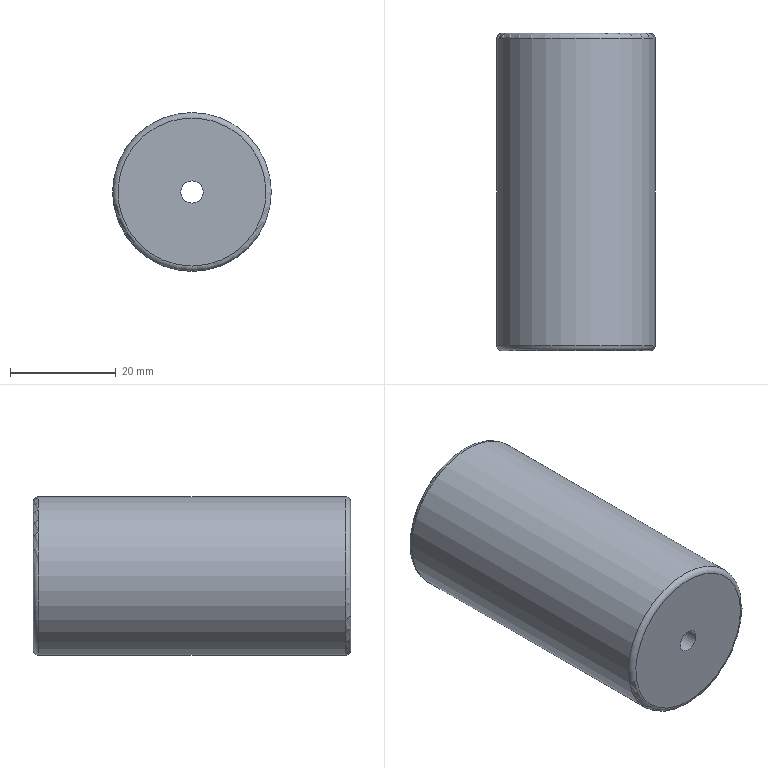Component | NX | 8_SLEEVE | 1 solid | 11 faces | box 30 x 60 x 30 mm | volume 28897 mm3 | plane 4 | cylinder 4 | torus 3 | commonest cylinder face diameters 30 x1 18 x1 20 x1 4.2 x1
STEP:
#1=CARTESIAN_POINT('',(0.,0.,0.));
#2=DIRECTION('',(0.,0.,1.));
#3=DIRECTION('',(1.,0.,0.));
#4=AXIS2_PLACEMENT_3D('',#1,#2,#3);
#5=CARTESIAN_POINT('',(-59.084,-92.206,-228.219));
#6=VERTEX_POINT('',#5);
#7=CARTESIAN_POINT('',(-59.084,-92.206,-238.219));
#8=DIRECTION('',(0.,-1.,0.));
#9=DIRECTION('',(0.,0.,1.));
#10=AXIS2_PLACEMENT_3D('',#7,#8,#9);
#11=CIRCLE('',#10,10.);
#12=CARTESIAN_POINT('',(-59.084,-92.206,-238.219));
#13=DIRECTION('',(0.,1.,0.));
#14=DIRECTION('',(0.,0.,1.));
#15=AXIS2_PLACEMENT_3D('',#12,#13,#14);
#16=PLANE('',#15);
#17=CARTESIAN_POINT('',(10.,0.));
#18=CARTESIAN_POINT('',(10.,-17.321));
#19=CARTESIAN_POINT('',(-5.,-8.66));
#20=CARTESIAN_POINT('',(-20.,-0.));
#21=CARTESIAN_POINT('',(-5.,8.66));
#22=CARTESIAN_POINT('',(10.,17.321));
#23=CARTESIAN_POINT('',(10.,0.));
#24=(BOUNDED_CURVE()B_SPLINE_CURVE(2,(#17,#18,#19,#20,#21,#22,#23),.UNSPECIFIED.,.T.,.F.)B_SPLINE_CURVE_WITH_KNOTS((1,2,2,2,2,1),(-2.094,0.,2.094,4.189,6.283,8.378),.UNSPECIFIED.)CURVE()GEOMETRIC_REPRESENTATION_ITEM()RATIONAL_B_SPLINE_CURVE((1.,0.5,1.,0.5,1.,0.5,1.))REPRESENTATION_ITEM(''));
#25=(GEOMETRIC_REPRESENTATION_CONTEXT(2)PARAMETRIC_REPRESENTATION_CONTEXT()REPRESENTATION_CONTEXT('',''));
#26=DEFINITIONAL_REPRESENTATION('',(#24),#25);
#27=PCURVE('',#16,#26);
#28=CARTESIAN_POINT('',(-59.084,-93.206,-238.219));
#29=DIRECTION('',(0.,1.,0.));
#30=DIRECTION('',(0.,0.,1.));
#31=AXIS2_PLACEMENT_3D('',#28,#29,#30);
#32=TOROIDAL_SURFACE('',#31,10.,1.);
#33=CARTESIAN_POINT('',(6.283,7.854));
#34=DIRECTION('',(-1.,0.));
#35=VECTOR('',#34,1.);
#36=LINE('',#33,#35);
#37=(GEOMETRIC_REPRESENTATION_CONTEXT(2)PARAMETRIC_REPRESENTATION_CONTEXT()REPRESENTATION_CONTEXT('',''));
#38=DEFINITIONAL_REPRESENTATION('',(#36),#37);
#39=PCURVE('',#32,#38);
#40=SURFACE_CURVE('',#11,(#27,#39),.PCURVE_S1.);
#41=EDGE_CURVE('',#6,#6,#40,.T.);
#42=ORIENTED_EDGE('',*,*,#41,.T.);
#43=EDGE_LOOP('',(#42));
#44=FACE_BOUND('',#43,.T.);
#45=CARTESIAN_POINT('',(-59.084,-92.206,-224.219));
#46=VERTEX_POINT('',#45);
#47=CARTESIAN_POINT('',(-59.084,-92.206,-238.219));
#48=DIRECTION('',(0.,1.,0.));
#49=DIRECTION('',(0.,0.,1.));
#50=AXIS2_PLACEMENT_3D('',#47,#48,#49);
#51=CIRCLE('',#50,14.);
#52=CARTESIAN_POINT('',(0.,0.));
#53=DIRECTION('',(1.,0.));
#54=AXIS2_PLACEMENT_2D('',#52,#53);
#55=CIRCLE('',#54,14.);
#56=(GEOMETRIC_REPRESENTATION_CONTEXT(2)PARAMETRIC_REPRESENTATION_CONTEXT()REPRESENTATION_CONTEXT('',''));
#57=DEFINITIONAL_REPRESENTATION('',(#55),#56);
#58=PCURVE('',#16,#57);
#59=CARTESIAN_POINT('',(-59.084,-93.206,-238.219));
#60=DIRECTION('',(0.,1.,0.));
#61=DIRECTION('',(0.,0.,1.));
#62=AXIS2_PLACEMENT_3D('',#59,#60,#61);
#63=TOROIDAL_SURFACE('',#62,14.,1.);
#64=CARTESIAN_POINT('',(0.,7.854));
#65=DIRECTION('',(1.,0.));
#66=VECTOR('',#65,1.);
#67=LINE('',#64,#66);
#68=(GEOMETRIC_REPRESENTATION_CONTEXT(2)PARAMETRIC_REPRESENTATION_CONTEXT()REPRESENTATION_CONTEXT('',''));
#69=DEFINITIONAL_REPRESENTATION('',(#67),#68);
#70=PCURVE('',#63,#69);
#71=SURFACE_CURVE('',#51,(#58,#70),.PCURVE_S1.);
#72=EDGE_CURVE('',#46,#46,#71,.T.);
#73=ORIENTED_EDGE('',*,*,#72,.T.);
#74=EDGE_LOOP('',(#73));
#75=FACE_BOUND('',#74,.T.);
#76=ADVANCED_FACE('',(#44,#75),#16,.T.);
#77=CARTESIAN_POINT('',(-59.084,-152.206,-252.219));
#78=VERTEX_POINT('',#77);
#79=CARTESIAN_POINT('',(-59.084,-152.206,-238.219));
#80=DIRECTION('',(0.,-1.,0.));
#81=DIRECTION('',(0.,0.,-1.));
#82=AXIS2_PLACEMENT_3D('',#79,#80,#81);
#83=CIRCLE('',#82,14.);
#84=CARTESIAN_POINT('',(-59.084,-152.206,-238.219));
#85=DIRECTION('',(0.,-1.,0.));
#86=DIRECTION('',(0.,0.,-1.));
#87=AXIS2_PLACEMENT_3D('',#84,#85,#86);
#88=PLANE('',#87);
#89=CARTESIAN_POINT('',(0.,0.));
#90=DIRECTION('',(1.,0.));
#91=AXIS2_PLACEMENT_2D('',#89,#90);
#92=CIRCLE('',#91,14.);
#93=(GEOMETRIC_REPRESENTATION_CONTEXT(2)PARAMETRIC_REPRESENTATION_CONTEXT()REPRESENTATION_CONTEXT('',''));
#94=DEFINITIONAL_REPRESENTATION('',(#92),#93);
#95=PCURVE('',#88,#94);
#96=CARTESIAN_POINT('',(-59.084,-151.206,-238.219));
#97=DIRECTION('',(0.,-1.,0.));
#98=DIRECTION('',(0.,0.,-1.));
#99=AXIS2_PLACEMENT_3D('',#96,#97,#98);
#100=TOROIDAL_SURFACE('',#99,14.,1.);
#101=CARTESIAN_POINT('',(0.,7.854));
#102=DIRECTION('',(1.,0.));
#103=VECTOR('',#102,1.);
#104=LINE('',#101,#103);
#105=(GEOMETRIC_REPRESENTATION_CONTEXT(2)PARAMETRIC_REPRESENTATION_CONTEXT()REPRESENTATION_CONTEXT('',''));
#106=DEFINITIONAL_REPRESENTATION('',(#104),#105);
#107=PCURVE('',#100,#106);
#108=SURFACE_CURVE('',#83,(#95,#107),.PCURVE_S1.);
#109=EDGE_CURVE('',#78,#78,#108,.T.);
#110=ORIENTED_EDGE('',*,*,#109,.T.);
#111=EDGE_LOOP('',(#110));
#112=FACE_BOUND('',#111,.T.);
#113=CARTESIAN_POINT('',(-59.084,-152.206,-236.119));
#114=VERTEX_POINT('',#113);
#115=CARTESIAN_POINT('',(-59.084,-152.206,-238.219));
#116=DIRECTION('',(0.,1.,0.));
#117=DIRECTION('',(0.,0.,1.));
#118=AXIS2_PLACEMENT_3D('',#115,#116,#117);
#119=CIRCLE('',#118,2.1);
#120=CARTESIAN_POINT('',(-2.1,0.));
#121=CARTESIAN_POINT('',(-2.1,3.637));
#122=CARTESIAN_POINT('',(1.05,1.819));
#123=CARTESIAN_POINT('',(4.2,0.));
#124=CARTESIAN_POINT('',(1.05,-1.819));
#125=CARTESIAN_POINT('',(-2.1,-3.637));
#126=CARTESIAN_POINT('',(-2.1,0.));
#127=(BOUNDED_CURVE()B_SPLINE_CURVE(2,(#120,#121,#122,#123,#124,#125,#126),.UNSPECIFIED.,.T.,.F.)B_SPLINE_CURVE_WITH_KNOTS((1,2,2,2,2,1),(-2.094,0.,2.094,4.189,6.283,8.378),.UNSPECIFIED.)CURVE()GEOMETRIC_REPRESENTATION_ITEM()RATIONAL_B_SPLINE_CURVE((1.,0.5,1.,0.5,1.,0.5,1.))REPRESENTATION_ITEM(''));
#128=(GEOMETRIC_REPRESENTATION_CONTEXT(2)PARAMETRIC_REPRESENTATION_CONTEXT()REPRESENTATION_CONTEXT('',''));
#129=DEFINITIONAL_REPRESENTATION('',(#127),#128);
#130=PCURVE('',#88,#129);
#131=CARTESIAN_POINT('',(-59.084,-152.206,-238.219));
#132=DIRECTION('',(0.,1.,0.));
#133=DIRECTION('',(0.,0.,1.));
#134=AXIS2_PLACEMENT_3D('',#131,#132,#133);
#135=CYLINDRICAL_SURFACE('',#134,2.1);
#136=CARTESIAN_POINT('',(0.,0.));
#137=DIRECTION('',(1.,0.));
#138=VECTOR('',#137,1.);
#139=LINE('',#136,#138);
#140=(GEOMETRIC_REPRESENTATION_CONTEXT(2)PARAMETRIC_REPRESENTATION_CONTEXT()REPRESENTATION_CONTEXT('',''));
#141=DEFINITIONAL_REPRESENTATION('',(#139),#140);
#142=PCURVE('',#135,#141);
#143=SURFACE_CURVE('',#119,(#130,#142),.PCURVE_S1.);
#144=EDGE_CURVE('',#114,#114,#143,.T.);
#145=ORIENTED_EDGE('',*,*,#144,.T.);
#146=EDGE_LOOP('',(#145));
#147=FACE_BOUND('',#146,.T.);
#148=ADVANCED_FACE('',(#112,#147),#88,.T.);
#149=CARTESIAN_POINT('',(-59.084,-93.206,-223.219));
#150=VERTEX_POINT('',#149);
#151=CARTESIAN_POINT('',(-59.084,-93.206,-238.219));
#152=DIRECTION('',(0.,-1.,0.));
#153=DIRECTION('',(0.,0.,1.));
#154=AXIS2_PLACEMENT_3D('',#151,#152,#153);
#155=CIRCLE('',#154,15.);
#156=CARTESIAN_POINT('',(-59.084,-152.206,-238.219));
#157=DIRECTION('',(0.,1.,0.));
#158=DIRECTION('',(0.,0.,1.));
#159=AXIS2_PLACEMENT_3D('',#156,#157,#158);
#160=CYLINDRICAL_SURFACE('',#159,15.);
#161=CARTESIAN_POINT('',(6.283,59.));
#162=DIRECTION('',(-1.,0.));
#163=VECTOR('',#162,1.);
#164=LINE('',#161,#163);
#165=(GEOMETRIC_REPRESENTATION_CONTEXT(2)PARAMETRIC_REPRESENTATION_CONTEXT()REPRESENTATION_CONTEXT('',''));
#166=DEFINITIONAL_REPRESENTATION('',(#164),#165);
#167=PCURVE('',#160,#166);
#168=CARTESIAN_POINT('',(6.283,6.283));
#169=DIRECTION('',(-1.,0.));
#170=VECTOR('',#169,1.);
#171=LINE('',#168,#170);
#172=(GEOMETRIC_REPRESENTATION_CONTEXT(2)PARAMETRIC_REPRESENTATION_CONTEXT()REPRESENTATION_CONTEXT('',''));
#173=DEFINITIONAL_REPRESENTATION('',(#171),#172);
#174=PCURVE('',#63,#173);
#175=SURFACE_CURVE('',#155,(#167,#174),.PCURVE_S1.);
#176=EDGE_CURVE('',#150,#150,#175,.T.);
#177=ORIENTED_EDGE('',*,*,#176,.T.);
#178=CARTESIAN_POINT('',(-59.084,-151.206,-223.219));
#179=VERTEX_POINT('',#178);
#180=CARTESIAN_POINT('',(-59.084,-151.206,-223.219));
#181=CARTESIAN_POINT('',(-59.084,-93.206,-223.219));
#182=B_SPLINE_CURVE_WITH_KNOTS('',1,(#180,#181),.UNSPECIFIED.,.F.,.F.,(2,2),(1.,59.),.PIECEWISE_BEZIER_KNOTS.);
#183=CARTESIAN_POINT('',(0.,0.));
#184=DIRECTION('',(0.,1.));
#185=VECTOR('',#184,1.);
#186=LINE('',#183,#185);
#187=(GEOMETRIC_REPRESENTATION_CONTEXT(2)PARAMETRIC_REPRESENTATION_CONTEXT()REPRESENTATION_CONTEXT('',''));
#188=DEFINITIONAL_REPRESENTATION('',(#186),#187);
#189=PCURVE('',#160,#188);
#190=CARTESIAN_POINT('',(6.283,0.));
#191=DIRECTION('',(0.,1.));
#192=VECTOR('',#191,1.);
#193=LINE('',#190,#192);
#194=(GEOMETRIC_REPRESENTATION_CONTEXT(2)PARAMETRIC_REPRESENTATION_CONTEXT()REPRESENTATION_CONTEXT('',''));
#195=DEFINITIONAL_REPRESENTATION('',(#193),#194);
#196=PCURVE('',#160,#195);
#197=SEAM_CURVE('',#182,(#189,#196),.PCURVE_S1.);
#198=EDGE_CURVE('',#179,#150,#197,.T.);
#199=ORIENTED_EDGE('',*,*,#198,.F.);
#200=CARTESIAN_POINT('',(-59.084,-151.206,-253.219));
#201=VERTEX_POINT('',#200);
#202=CARTESIAN_POINT('',(-59.084,-151.206,-238.219));
#203=DIRECTION('',(0.,1.,0.));
#204=DIRECTION('',(0.,0.,-1.));
#205=AXIS2_PLACEMENT_3D('',#202,#203,#204);
#206=CIRCLE('',#205,15.);
#207=CARTESIAN_POINT('',(-3.142,1.));
#208=DIRECTION('',(1.,0.));
#209=VECTOR('',#208,1.);
#210=LINE('',#207,#209);
#211=(GEOMETRIC_REPRESENTATION_CONTEXT(2)PARAMETRIC_REPRESENTATION_CONTEXT()REPRESENTATION_CONTEXT('',''));
#212=DEFINITIONAL_REPRESENTATION('',(#210),#211);
#213=PCURVE('',#160,#212);
#214=CARTESIAN_POINT('',(6.283,6.283));
#215=DIRECTION('',(-1.,0.));
#216=VECTOR('',#215,1.);
#217=LINE('',#214,#216);
#218=(GEOMETRIC_REPRESENTATION_CONTEXT(2)PARAMETRIC_REPRESENTATION_CONTEXT()REPRESENTATION_CONTEXT('',''));
#219=DEFINITIONAL_REPRESENTATION('',(#217),#218);
#220=PCURVE('',#100,#219);
#221=SURFACE_CURVE('',#206,(#213,#220),.PCURVE_S1.);
#222=EDGE_CURVE('',#179,#201,#221,.T.);
#223=ORIENTED_EDGE('',*,*,#222,.T.);
#224=CARTESIAN_POINT('',(-59.084,-151.206,-238.219));
#225=DIRECTION('',(0.,1.,0.));
#226=DIRECTION('',(0.,0.,-1.));
#227=AXIS2_PLACEMENT_3D('',#224,#225,#226);
#228=CIRCLE('',#227,15.);
#229=CARTESIAN_POINT('',(3.142,1.));
#230=DIRECTION('',(1.,0.));
#231=VECTOR('',#230,1.);
#232=LINE('',#229,#231);
#233=(GEOMETRIC_REPRESENTATION_CONTEXT(2)PARAMETRIC_REPRESENTATION_CONTEXT()REPRESENTATION_CONTEXT('',''));
#234=DEFINITIONAL_REPRESENTATION('',(#232),#233);
#235=PCURVE('',#160,#234);
#236=CARTESIAN_POINT('',(6.283,6.283));
#237=DIRECTION('',(-1.,0.));
#238=VECTOR('',#237,1.);
#239=LINE('',#236,#238);
#240=(GEOMETRIC_REPRESENTATION_CONTEXT(2)PARAMETRIC_REPRESENTATION_CONTEXT()REPRESENTATION_CONTEXT('',''));
#241=DEFINITIONAL_REPRESENTATION('',(#239),#240);
#242=PCURVE('',#100,#241);
#243=SURFACE_CURVE('',#228,(#235,#242),.PCURVE_S1.);
#244=EDGE_CURVE('',#201,#179,#243,.T.);
#245=ORIENTED_EDGE('',*,*,#244,.T.);
#246=ORIENTED_EDGE('',*,*,#198,.T.);
#247=EDGE_LOOP('',(#177,#199,#223,#245,#246));
#248=FACE_BOUND('',#247,.T.);
#249=ADVANCED_FACE('',(#248),#160,.T.);
#250=CARTESIAN_POINT('',(-59.084,-93.206,-229.219));
#251=VERTEX_POINT('',#250);
#252=CARTESIAN_POINT('',(-59.084,-93.206,-238.219));
#253=DIRECTION('',(0.,1.,0.));
#254=DIRECTION('',(0.,0.,1.));
#255=AXIS2_PLACEMENT_3D('',#252,#253,#254);
#256=CIRCLE('',#255,9.);
#257=CARTESIAN_POINT('',(-59.084,-92.206,-238.219));
#258=DIRECTION('',(0.,-1.,0.));
#259=DIRECTION('',(0.,0.,1.));
#260=AXIS2_PLACEMENT_3D('',#257,#258,#259);
#261=CYLINDRICAL_SURFACE('',#260,9.);
#262=CARTESIAN_POINT('',(6.283,1.));
#263=DIRECTION('',(-1.,0.));
#264=VECTOR('',#263,1.);
#265=LINE('',#262,#264);
#266=(GEOMETRIC_REPRESENTATION_CONTEXT(2)PARAMETRIC_REPRESENTATION_CONTEXT()REPRESENTATION_CONTEXT('',''));
#267=DEFINITIONAL_REPRESENTATION('',(#265),#266);
#268=PCURVE('',#261,#267);
#269=CARTESIAN_POINT('',(0.,9.425));
#270=DIRECTION('',(1.,0.));
#271=VECTOR('',#270,1.);
#272=LINE('',#269,#271);
#273=(GEOMETRIC_REPRESENTATION_CONTEXT(2)PARAMETRIC_REPRESENTATION_CONTEXT()REPRESENTATION_CONTEXT('',''));
#274=DEFINITIONAL_REPRESENTATION('',(#272),#273);
#275=PCURVE('',#32,#274);
#276=SURFACE_CURVE('',#256,(#268,#275),.PCURVE_S1.);
#277=EDGE_CURVE('',#251,#251,#276,.T.);
#278=ORIENTED_EDGE('',*,*,#277,.F.);
#279=CARTESIAN_POINT('',(-59.084,-142.206,-229.219));
#280=VERTEX_POINT('',#279);
#281=CARTESIAN_POINT('',(-59.084,-93.206,-229.219));
#282=CARTESIAN_POINT('',(-59.084,-142.206,-229.219));
#283=B_SPLINE_CURVE_WITH_KNOTS('',1,(#281,#282),.UNSPECIFIED.,.F.,.F.,(2,2),(1.,50.),.PIECEWISE_BEZIER_KNOTS.);
#284=CARTESIAN_POINT('',(6.283,0.));
#285=DIRECTION('',(0.,1.));
#286=VECTOR('',#285,1.);
#287=LINE('',#284,#286);
#288=(GEOMETRIC_REPRESENTATION_CONTEXT(2)PARAMETRIC_REPRESENTATION_CONTEXT()REPRESENTATION_CONTEXT('',''));
#289=DEFINITIONAL_REPRESENTATION('',(#287),#288);
#290=PCURVE('',#261,#289);
#291=CARTESIAN_POINT('',(0.,0.));
#292=DIRECTION('',(0.,1.));
#293=VECTOR('',#292,1.);
#294=LINE('',#291,#293);
#295=(GEOMETRIC_REPRESENTATION_CONTEXT(2)PARAMETRIC_REPRESENTATION_CONTEXT()REPRESENTATION_CONTEXT('',''));
#296=DEFINITIONAL_REPRESENTATION('',(#294),#295);
#297=PCURVE('',#261,#296);
#298=SEAM_CURVE('',#283,(#290,#297),.PCURVE_S1.);
#299=EDGE_CURVE('',#251,#280,#298,.T.);
#300=ORIENTED_EDGE('',*,*,#299,.T.);
#301=CARTESIAN_POINT('',(-59.084,-142.206,-238.219));
#302=DIRECTION('',(0.,-1.,0.));
#303=DIRECTION('',(0.,0.,1.));
#304=AXIS2_PLACEMENT_3D('',#301,#302,#303);
#305=CIRCLE('',#304,9.);
#306=CARTESIAN_POINT('',(0.,50.));
#307=DIRECTION('',(1.,0.));
#308=VECTOR('',#307,1.);
#309=LINE('',#306,#308);
#310=(GEOMETRIC_REPRESENTATION_CONTEXT(2)PARAMETRIC_REPRESENTATION_CONTEXT()REPRESENTATION_CONTEXT('',''));
#311=DEFINITIONAL_REPRESENTATION('',(#309),#310);
#312=PCURVE('',#261,#311);
#313=CARTESIAN_POINT('',(-59.084,-142.206,-238.219));
#314=DIRECTION('',(0.,1.,0.));
#315=DIRECTION('',(0.,0.,1.));
#316=AXIS2_PLACEMENT_3D('',#313,#314,#315);
#317=PLANE('',#316);
#318=CARTESIAN_POINT('',(9.,0.));
#319=CARTESIAN_POINT('',(9.,-15.588));
#320=CARTESIAN_POINT('',(-4.5,-7.794));
#321=CARTESIAN_POINT('',(-18.,-0.));
#322=CARTESIAN_POINT('',(-4.5,7.794));
#323=CARTESIAN_POINT('',(9.,15.588));
#324=CARTESIAN_POINT('',(9.,0.));
#325=(BOUNDED_CURVE()B_SPLINE_CURVE(2,(#318,#319,#320,#321,#322,#323,#324),.UNSPECIFIED.,.T.,.F.)B_SPLINE_CURVE_WITH_KNOTS((1,2,2,2,2,1),(-2.094,0.,2.094,4.189,6.283,8.378),.UNSPECIFIED.)CURVE()GEOMETRIC_REPRESENTATION_ITEM()RATIONAL_B_SPLINE_CURVE((1.,0.5,1.,0.5,1.,0.5,1.))REPRESENTATION_ITEM(''));
#326=(GEOMETRIC_REPRESENTATION_CONTEXT(2)PARAMETRIC_REPRESENTATION_CONTEXT()REPRESENTATION_CONTEXT('',''));
#327=DEFINITIONAL_REPRESENTATION('',(#325),#326);
#328=PCURVE('',#317,#327);
#329=SURFACE_CURVE('',#305,(#312,#328),.PCURVE_S1.);
#330=EDGE_CURVE('',#280,#280,#329,.T.);
#331=ORIENTED_EDGE('',*,*,#330,.F.);
#332=ORIENTED_EDGE('',*,*,#299,.F.);
#333=EDGE_LOOP('',(#278,#300,#331,#332));
#334=FACE_BOUND('',#333,.F.);
#335=ADVANCED_FACE('',(#334),#261,.F.);
#336=CARTESIAN_POINT('',(-59.084,-142.206,-228.219));
#337=VERTEX_POINT('',#336);
#338=CARTESIAN_POINT('',(-59.084,-142.206,-238.219));
#339=DIRECTION('',(0.,1.,0.));
#340=DIRECTION('',(0.,0.,1.));
#341=AXIS2_PLACEMENT_3D('',#338,#339,#340);
#342=CIRCLE('',#341,10.);
#343=CARTESIAN_POINT('',(0.,0.));
#344=DIRECTION('',(1.,0.));
#345=AXIS2_PLACEMENT_2D('',#343,#344);
#346=CIRCLE('',#345,10.);
#347=(GEOMETRIC_REPRESENTATION_CONTEXT(2)PARAMETRIC_REPRESENTATION_CONTEXT()REPRESENTATION_CONTEXT('',''));
#348=DEFINITIONAL_REPRESENTATION('',(#346),#347);
#349=PCURVE('',#317,#348);
#350=CARTESIAN_POINT('',(-59.084,-142.206,-238.219));
#351=DIRECTION('',(0.,-1.,0.));
#352=DIRECTION('',(0.,0.,1.));
#353=AXIS2_PLACEMENT_3D('',#350,#351,#352);
#354=CYLINDRICAL_SURFACE('',#353,10.);
#355=CARTESIAN_POINT('',(6.283,0.));
#356=DIRECTION('',(-1.,0.));
#357=VECTOR('',#356,1.);
#358=LINE('',#355,#357);
#359=(GEOMETRIC_REPRESENTATION_CONTEXT(2)PARAMETRIC_REPRESENTATION_CONTEXT()REPRESENTATION_CONTEXT('',''));
#360=DEFINITIONAL_REPRESENTATION('',(#358),#359);
#361=PCURVE('',#354,#360);
#362=SURFACE_CURVE('',#342,(#349,#361),.PCURVE_S1.);
#363=EDGE_CURVE('',#337,#337,#362,.T.);
#364=ORIENTED_EDGE('',*,*,#363,.F.);
#365=EDGE_LOOP('',(#364));
#366=FACE_BOUND('',#365,.T.);
#367=ORIENTED_EDGE('',*,*,#330,.F.);
#368=EDGE_LOOP('',(#367));
#369=FACE_BOUND('',#368,.T.);
#370=ADVANCED_FACE('',(#366,#369),#317,.F.);
#371=CARTESIAN_POINT('',(-59.084,-144.206,-240.319));
#372=VERTEX_POINT('',#371);
#373=CARTESIAN_POINT('',(-59.084,-144.206,-236.119));
#374=VERTEX_POINT('',#373);
#375=CARTESIAN_POINT('',(-59.084,-144.206,-238.219));
#376=DIRECTION('',(0.,-1.,0.));
#377=DIRECTION('',(0.,0.,-1.));
#378=AXIS2_PLACEMENT_3D('',#375,#376,#377);
#379=CIRCLE('',#378,2.1);
#380=CARTESIAN_POINT('',(-59.084,-144.206,-238.219));
#381=DIRECTION('',(0.,-1.,0.));
#382=DIRECTION('',(0.,0.,-1.));
#383=AXIS2_PLACEMENT_3D('',#380,#381,#382);
#384=PLANE('',#383);
#385=CARTESIAN_POINT('',(0.,0.));
#386=DIRECTION('',(1.,0.));
#387=AXIS2_PLACEMENT_2D('',#385,#386);
#388=CIRCLE('',#387,2.1);
#389=(GEOMETRIC_REPRESENTATION_CONTEXT(2)PARAMETRIC_REPRESENTATION_CONTEXT()REPRESENTATION_CONTEXT('',''));
#390=DEFINITIONAL_REPRESENTATION('',(#388),#389);
#391=PCURVE('',#384,#390);
#392=CARTESIAN_POINT('',(3.142,8.));
#393=DIRECTION('',(-1.,0.));
#394=VECTOR('',#393,1.);
#395=LINE('',#392,#394);
#396=(GEOMETRIC_REPRESENTATION_CONTEXT(2)PARAMETRIC_REPRESENTATION_CONTEXT()REPRESENTATION_CONTEXT('',''));
#397=DEFINITIONAL_REPRESENTATION('',(#395),#396);
#398=PCURVE('',#135,#397);
#399=SURFACE_CURVE('',#379,(#391,#398),.PCURVE_S1.);
#400=EDGE_CURVE('',#372,#374,#399,.T.);
#401=ORIENTED_EDGE('',*,*,#400,.T.);
#402=CARTESIAN_POINT('',(-59.084,-144.206,-238.219));
#403=DIRECTION('',(0.,-1.,0.));
#404=DIRECTION('',(0.,0.,-1.));
#405=AXIS2_PLACEMENT_3D('',#402,#403,#404);
#406=CIRCLE('',#405,2.1);
#407=CARTESIAN_POINT('',(0.,0.));
#408=DIRECTION('',(1.,0.));
#409=AXIS2_PLACEMENT_2D('',#407,#408);
#410=CIRCLE('',#409,2.1);
#411=(GEOMETRIC_REPRESENTATION_CONTEXT(2)PARAMETRIC_REPRESENTATION_CONTEXT()REPRESENTATION_CONTEXT('',''));
#412=DEFINITIONAL_REPRESENTATION('',(#410),#411);
#413=PCURVE('',#384,#412);
#414=CARTESIAN_POINT('',(9.425,8.));
#415=DIRECTION('',(-1.,0.));
#416=VECTOR('',#415,1.);
#417=LINE('',#414,#416);
#418=(GEOMETRIC_REPRESENTATION_CONTEXT(2)PARAMETRIC_REPRESENTATION_CONTEXT()REPRESENTATION_CONTEXT('',''));
#419=DEFINITIONAL_REPRESENTATION('',(#417),#418);
#420=PCURVE('',#135,#419);
#421=SURFACE_CURVE('',#406,(#413,#420),.PCURVE_S1.);
#422=EDGE_CURVE('',#374,#372,#421,.T.);
#423=ORIENTED_EDGE('',*,*,#422,.T.);
#424=EDGE_LOOP('',(#401,#423));
#425=FACE_BOUND('',#424,.T.);
#426=CARTESIAN_POINT('',(-59.084,-144.206,-228.219));
#427=VERTEX_POINT('',#426);
#428=CARTESIAN_POINT('',(-59.084,-144.206,-238.219));
#429=DIRECTION('',(0.,-1.,0.));
#430=DIRECTION('',(0.,0.,1.));
#431=AXIS2_PLACEMENT_3D('',#428,#429,#430);
#432=CIRCLE('',#431,10.);
#433=CARTESIAN_POINT('',(0.,0.));
#434=DIRECTION('',(-1.,0.));
#435=AXIS2_PLACEMENT_2D('',#433,#434);
#436=CIRCLE('',#435,10.);
#437=(GEOMETRIC_REPRESENTATION_CONTEXT(2)PARAMETRIC_REPRESENTATION_CONTEXT()REPRESENTATION_CONTEXT('',''));
#438=DEFINITIONAL_REPRESENTATION('',(#436),#437);
#439=PCURVE('',#384,#438);
#440=CARTESIAN_POINT('',(0.,2.));
#441=DIRECTION('',(1.,0.));
#442=VECTOR('',#441,1.);
#443=LINE('',#440,#442);
#444=(GEOMETRIC_REPRESENTATION_CONTEXT(2)PARAMETRIC_REPRESENTATION_CONTEXT()REPRESENTATION_CONTEXT('',''));
#445=DEFINITIONAL_REPRESENTATION('',(#443),#444);
#446=PCURVE('',#354,#445);
#447=SURFACE_CURVE('',#432,(#439,#446),.PCURVE_S1.);
#448=EDGE_CURVE('',#427,#427,#447,.T.);
#449=ORIENTED_EDGE('',*,*,#448,.F.);
#450=EDGE_LOOP('',(#449));
#451=FACE_BOUND('',#450,.T.);
#452=ADVANCED_FACE('',(#425,#451),#384,.F.);
#453=ORIENTED_EDGE('',*,*,#448,.F.);
#454=CARTESIAN_POINT('',(-59.084,-142.206,-228.219));
#455=CARTESIAN_POINT('',(-59.084,-144.206,-228.219));
#456=B_SPLINE_CURVE_WITH_KNOTS('',1,(#454,#455),.UNSPECIFIED.,.F.,.F.,(2,2),(0.,2.),.PIECEWISE_BEZIER_KNOTS.);
#457=CARTESIAN_POINT('',(0.,0.));
#458=DIRECTION('',(0.,1.));
#459=VECTOR('',#458,1.);
#460=LINE('',#457,#459);
#461=(GEOMETRIC_REPRESENTATION_CONTEXT(2)PARAMETRIC_REPRESENTATION_CONTEXT()REPRESENTATION_CONTEXT('',''));
#462=DEFINITIONAL_REPRESENTATION('',(#460),#461);
#463=PCURVE('',#354,#462);
#464=CARTESIAN_POINT('',(6.283,0.));
#465=DIRECTION('',(0.,1.));
#466=VECTOR('',#465,1.);
#467=LINE('',#464,#466);
#468=(GEOMETRIC_REPRESENTATION_CONTEXT(2)PARAMETRIC_REPRESENTATION_CONTEXT()REPRESENTATION_CONTEXT('',''));
#469=DEFINITIONAL_REPRESENTATION('',(#467),#468);
#470=PCURVE('',#354,#469);
#471=SEAM_CURVE('',#456,(#463,#470),.PCURVE_S1.);
#472=EDGE_CURVE('',#337,#427,#471,.T.);
#473=ORIENTED_EDGE('',*,*,#472,.F.);
#474=ORIENTED_EDGE('',*,*,#363,.F.);
#475=ORIENTED_EDGE('',*,*,#472,.T.);
#476=EDGE_LOOP('',(#453,#473,#474,#475));
#477=FACE_BOUND('',#476,.F.);
#478=ADVANCED_FACE('',(#477),#354,.F.);
#479=ORIENTED_EDGE('',*,*,#144,.T.);
#480=CARTESIAN_POINT('',(-59.084,-152.206,-236.119));
#481=CARTESIAN_POINT('',(-59.084,-144.206,-236.119));
#482=B_SPLINE_CURVE_WITH_KNOTS('',1,(#480,#481),.UNSPECIFIED.,.F.,.F.,(2,2),(0.,8.),.PIECEWISE_BEZIER_KNOTS.);
#483=CARTESIAN_POINT('',(6.283,0.));
#484=DIRECTION('',(0.,1.));
#485=VECTOR('',#484,1.);
#486=LINE('',#483,#485);
#487=(GEOMETRIC_REPRESENTATION_CONTEXT(2)PARAMETRIC_REPRESENTATION_CONTEXT()REPRESENTATION_CONTEXT('',''));
#488=DEFINITIONAL_REPRESENTATION('',(#486),#487);
#489=PCURVE('',#135,#488);
#490=CARTESIAN_POINT('',(0.,0.));
#491=DIRECTION('',(0.,1.));
#492=VECTOR('',#491,1.);
#493=LINE('',#490,#492);
#494=(GEOMETRIC_REPRESENTATION_CONTEXT(2)PARAMETRIC_REPRESENTATION_CONTEXT()REPRESENTATION_CONTEXT('',''));
#495=DEFINITIONAL_REPRESENTATION('',(#493),#494);
#496=PCURVE('',#135,#495);
#497=SEAM_CURVE('',#482,(#489,#496),.PCURVE_S1.);
#498=EDGE_CURVE('',#114,#374,#497,.T.);
#499=ORIENTED_EDGE('',*,*,#498,.T.);
#500=ORIENTED_EDGE('',*,*,#422,.T.);
#501=ORIENTED_EDGE('',*,*,#400,.T.);
#502=ORIENTED_EDGE('',*,*,#498,.F.);
#503=EDGE_LOOP('',(#479,#499,#500,#501,#502));
#504=FACE_BOUND('',#503,.F.);
#505=ADVANCED_FACE('',(#504),#135,.F.);
#506=ORIENTED_EDGE('',*,*,#277,.F.);
#507=CARTESIAN_POINT('',(-59.084,-92.206,-228.219));
#508=CARTESIAN_POINT('',(-59.084,-92.206,-228.486));
#509=CARTESIAN_POINT('',(-59.084,-92.291,-228.747));
#510=CARTESIAN_POINT('',(-59.084,-92.454,-228.971));
#511=CARTESIAN_POINT('',(-59.084,-92.679,-229.134));
#512=CARTESIAN_POINT('',(-59.084,-92.939,-229.219));
#513=CARTESIAN_POINT('',(-59.084,-93.206,-229.219));
#514=(BOUNDED_CURVE()B_SPLINE_CURVE(6,(#507,#508,#509,#510,#511,#512,#513),.UNSPECIFIED.,.F.,.F.)B_SPLINE_CURVE_WITH_KNOTS((7,7),(1.571,3.142),.PIECEWISE_BEZIER_KNOTS.)CURVE()GEOMETRIC_REPRESENTATION_ITEM()RATIONAL_B_SPLINE_CURVE((1.031,1.01,0.9979,0.994,0.9979,1.01,1.031))REPRESENTATION_ITEM(''));
#515=CARTESIAN_POINT('',(0.,6.283));
#516=DIRECTION('',(0.,1.));
#517=VECTOR('',#516,1.);
#518=LINE('',#515,#517);
#519=(GEOMETRIC_REPRESENTATION_CONTEXT(2)PARAMETRIC_REPRESENTATION_CONTEXT()REPRESENTATION_CONTEXT('',''));
#520=DEFINITIONAL_REPRESENTATION('',(#518),#519);
#521=PCURVE('',#32,#520);
#522=CARTESIAN_POINT('',(6.283,6.283));
#523=DIRECTION('',(0.,1.));
#524=VECTOR('',#523,1.);
#525=LINE('',#522,#524);
#526=(GEOMETRIC_REPRESENTATION_CONTEXT(2)PARAMETRIC_REPRESENTATION_CONTEXT()REPRESENTATION_CONTEXT('',''));
#527=DEFINITIONAL_REPRESENTATION('',(#525),#526);
#528=PCURVE('',#32,#527);
#529=SEAM_CURVE('',#514,(#521,#528),.PCURVE_S1.);
#530=EDGE_CURVE('',#6,#251,#529,.T.);
#531=ORIENTED_EDGE('',*,*,#530,.F.);
#532=ORIENTED_EDGE('',*,*,#41,.F.);
#533=ORIENTED_EDGE('',*,*,#530,.T.);
#534=EDGE_LOOP('',(#506,#531,#532,#533));
#535=FACE_BOUND('',#534,.T.);
#536=ADVANCED_FACE('',(#535),#32,.T.);
#537=ORIENTED_EDGE('',*,*,#72,.F.);
#538=CARTESIAN_POINT('',(-59.084,-93.206,-223.219));
#539=CARTESIAN_POINT('',(-59.084,-92.939,-223.219));
#540=CARTESIAN_POINT('',(-59.084,-92.679,-223.304));
#541=CARTESIAN_POINT('',(-59.084,-92.454,-223.467));
#542=CARTESIAN_POINT('',(-59.084,-92.291,-223.691));
#543=CARTESIAN_POINT('',(-59.084,-92.206,-223.952));
#544=CARTESIAN_POINT('',(-59.084,-92.206,-224.219));
#545=(BOUNDED_CURVE()B_SPLINE_CURVE(6,(#538,#539,#540,#541,#542,#543,#544),.UNSPECIFIED.,.F.,.F.)B_SPLINE_CURVE_WITH_KNOTS((7,7),(0.,1.571),.PIECEWISE_BEZIER_KNOTS.)CURVE()GEOMETRIC_REPRESENTATION_ITEM()RATIONAL_B_SPLINE_CURVE((1.031,1.01,0.9979,0.994,0.9979,1.01,1.031))REPRESENTATION_ITEM(''));
#546=CARTESIAN_POINT('',(0.,6.283));
#547=DIRECTION('',(0.,1.));
#548=VECTOR('',#547,1.);
#549=LINE('',#546,#548);
#550=(GEOMETRIC_REPRESENTATION_CONTEXT(2)PARAMETRIC_REPRESENTATION_CONTEXT()REPRESENTATION_CONTEXT('',''));
#551=DEFINITIONAL_REPRESENTATION('',(#549),#550);
#552=PCURVE('',#63,#551);
#553=CARTESIAN_POINT('',(6.283,6.283));
#554=DIRECTION('',(0.,1.));
#555=VECTOR('',#554,1.);
#556=LINE('',#553,#555);
#557=(GEOMETRIC_REPRESENTATION_CONTEXT(2)PARAMETRIC_REPRESENTATION_CONTEXT()REPRESENTATION_CONTEXT('',''));
#558=DEFINITIONAL_REPRESENTATION('',(#556),#557);
#559=PCURVE('',#63,#558);
#560=SEAM_CURVE('',#545,(#552,#559),.PCURVE_S1.);
#561=EDGE_CURVE('',#150,#46,#560,.T.);
#562=ORIENTED_EDGE('',*,*,#561,.F.);
#563=ORIENTED_EDGE('',*,*,#176,.F.);
#564=ORIENTED_EDGE('',*,*,#561,.T.);
#565=EDGE_LOOP('',(#537,#562,#563,#564));
#566=FACE_BOUND('',#565,.T.);
#567=ADVANCED_FACE('',(#566),#63,.T.);
#568=ORIENTED_EDGE('',*,*,#109,.F.);
#569=CARTESIAN_POINT('',(-59.084,-151.206,-253.219));
#570=CARTESIAN_POINT('',(-59.084,-151.474,-253.219));
#571=CARTESIAN_POINT('',(-59.084,-151.734,-253.134));
#572=CARTESIAN_POINT('',(-59.084,-151.958,-252.971));
#573=CARTESIAN_POINT('',(-59.084,-152.121,-252.747));
#574=CARTESIAN_POINT('',(-59.084,-152.206,-252.486));
#575=CARTESIAN_POINT('',(-59.084,-152.206,-252.219));
#576=(BOUNDED_CURVE()B_SPLINE_CURVE(6,(#569,#570,#571,#572,#573,#574,#575),.UNSPECIFIED.,.F.,.F.)B_SPLINE_CURVE_WITH_KNOTS((7,7),(0.,1.571),.PIECEWISE_BEZIER_KNOTS.)CURVE()GEOMETRIC_REPRESENTATION_ITEM()RATIONAL_B_SPLINE_CURVE((1.031,1.01,0.9979,0.994,0.9979,1.01,1.031))REPRESENTATION_ITEM(''));
#577=CARTESIAN_POINT('',(0.,6.283));
#578=DIRECTION('',(0.,1.));
#579=VECTOR('',#578,1.);
#580=LINE('',#577,#579);
#581=(GEOMETRIC_REPRESENTATION_CONTEXT(2)PARAMETRIC_REPRESENTATION_CONTEXT()REPRESENTATION_CONTEXT('',''));
#582=DEFINITIONAL_REPRESENTATION('',(#580),#581);
#583=PCURVE('',#100,#582);
#584=CARTESIAN_POINT('',(6.283,6.283));
#585=DIRECTION('',(0.,1.));
#586=VECTOR('',#585,1.);
#587=LINE('',#584,#586);
#588=(GEOMETRIC_REPRESENTATION_CONTEXT(2)PARAMETRIC_REPRESENTATION_CONTEXT()REPRESENTATION_CONTEXT('',''));
#589=DEFINITIONAL_REPRESENTATION('',(#587),#588);
#590=PCURVE('',#100,#589);
#591=SEAM_CURVE('',#576,(#583,#590),.PCURVE_S1.);
#592=EDGE_CURVE('',#201,#78,#591,.T.);
#593=ORIENTED_EDGE('',*,*,#592,.F.);
#594=ORIENTED_EDGE('',*,*,#222,.F.);
#595=ORIENTED_EDGE('',*,*,#244,.F.);
#596=ORIENTED_EDGE('',*,*,#592,.T.);
#597=EDGE_LOOP('',(#568,#593,#594,#595,#596));
#598=FACE_BOUND('',#597,.T.);
#599=ADVANCED_FACE('',(#598),#100,.T.);
#600=CLOSED_SHELL('',(#76,#148,#249,#335,#370,#452,#478,#505,#536,#567,#599));
#601=MANIFOLD_SOLID_BREP('',#600);
#602=(LENGTH_UNIT()NAMED_UNIT(*)SI_UNIT(.MILLI.,.METRE.));
#603=UNCERTAINTY_MEASURE_WITH_UNIT(LENGTH_MEASURE(0.00001),#602,'','');
#604=(NAMED_UNIT(*)PLANE_ANGLE_UNIT()SI_UNIT($,.RADIAN.));
#605=(NAMED_UNIT(*)SI_UNIT($,.STERADIAN.)SOLID_ANGLE_UNIT());
#606=(GEOMETRIC_REPRESENTATION_CONTEXT(3)GLOBAL_UNCERTAINTY_ASSIGNED_CONTEXT((#603))GLOBAL_UNIT_ASSIGNED_CONTEXT((#602,#604,#605))REPRESENTATION_CONTEXT('',''));
#607=ADVANCED_BREP_SHAPE_REPRESENTATION('',(#4,#601),#606);